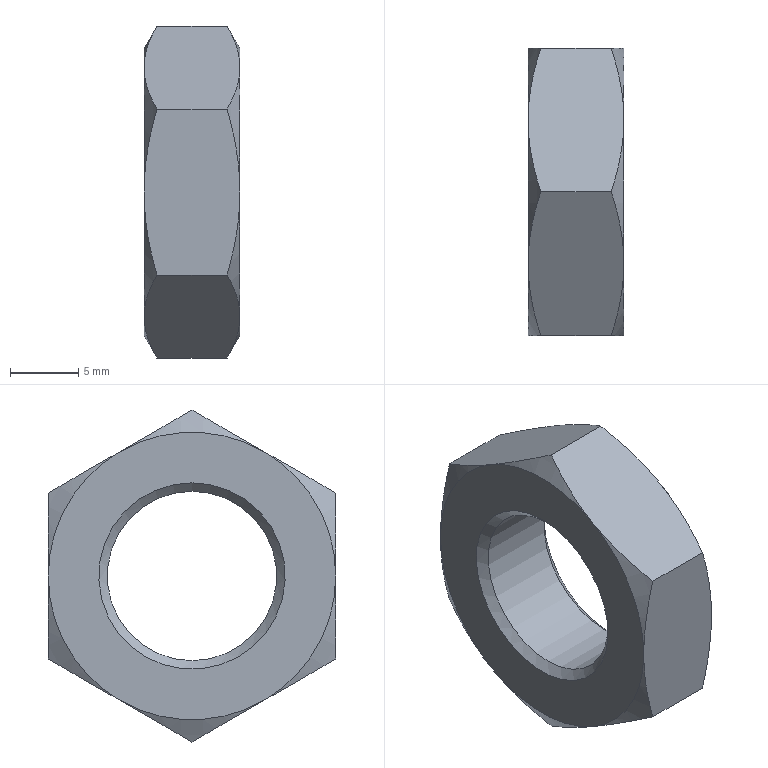Component | NX | GB-T6172_1-2000_M14X2 | 1 solid | 23 faces | volume 1795 mm3 | cone 14 | plane 8 | cylinder 1 | commonest cylinder face diameters 12.376 x1